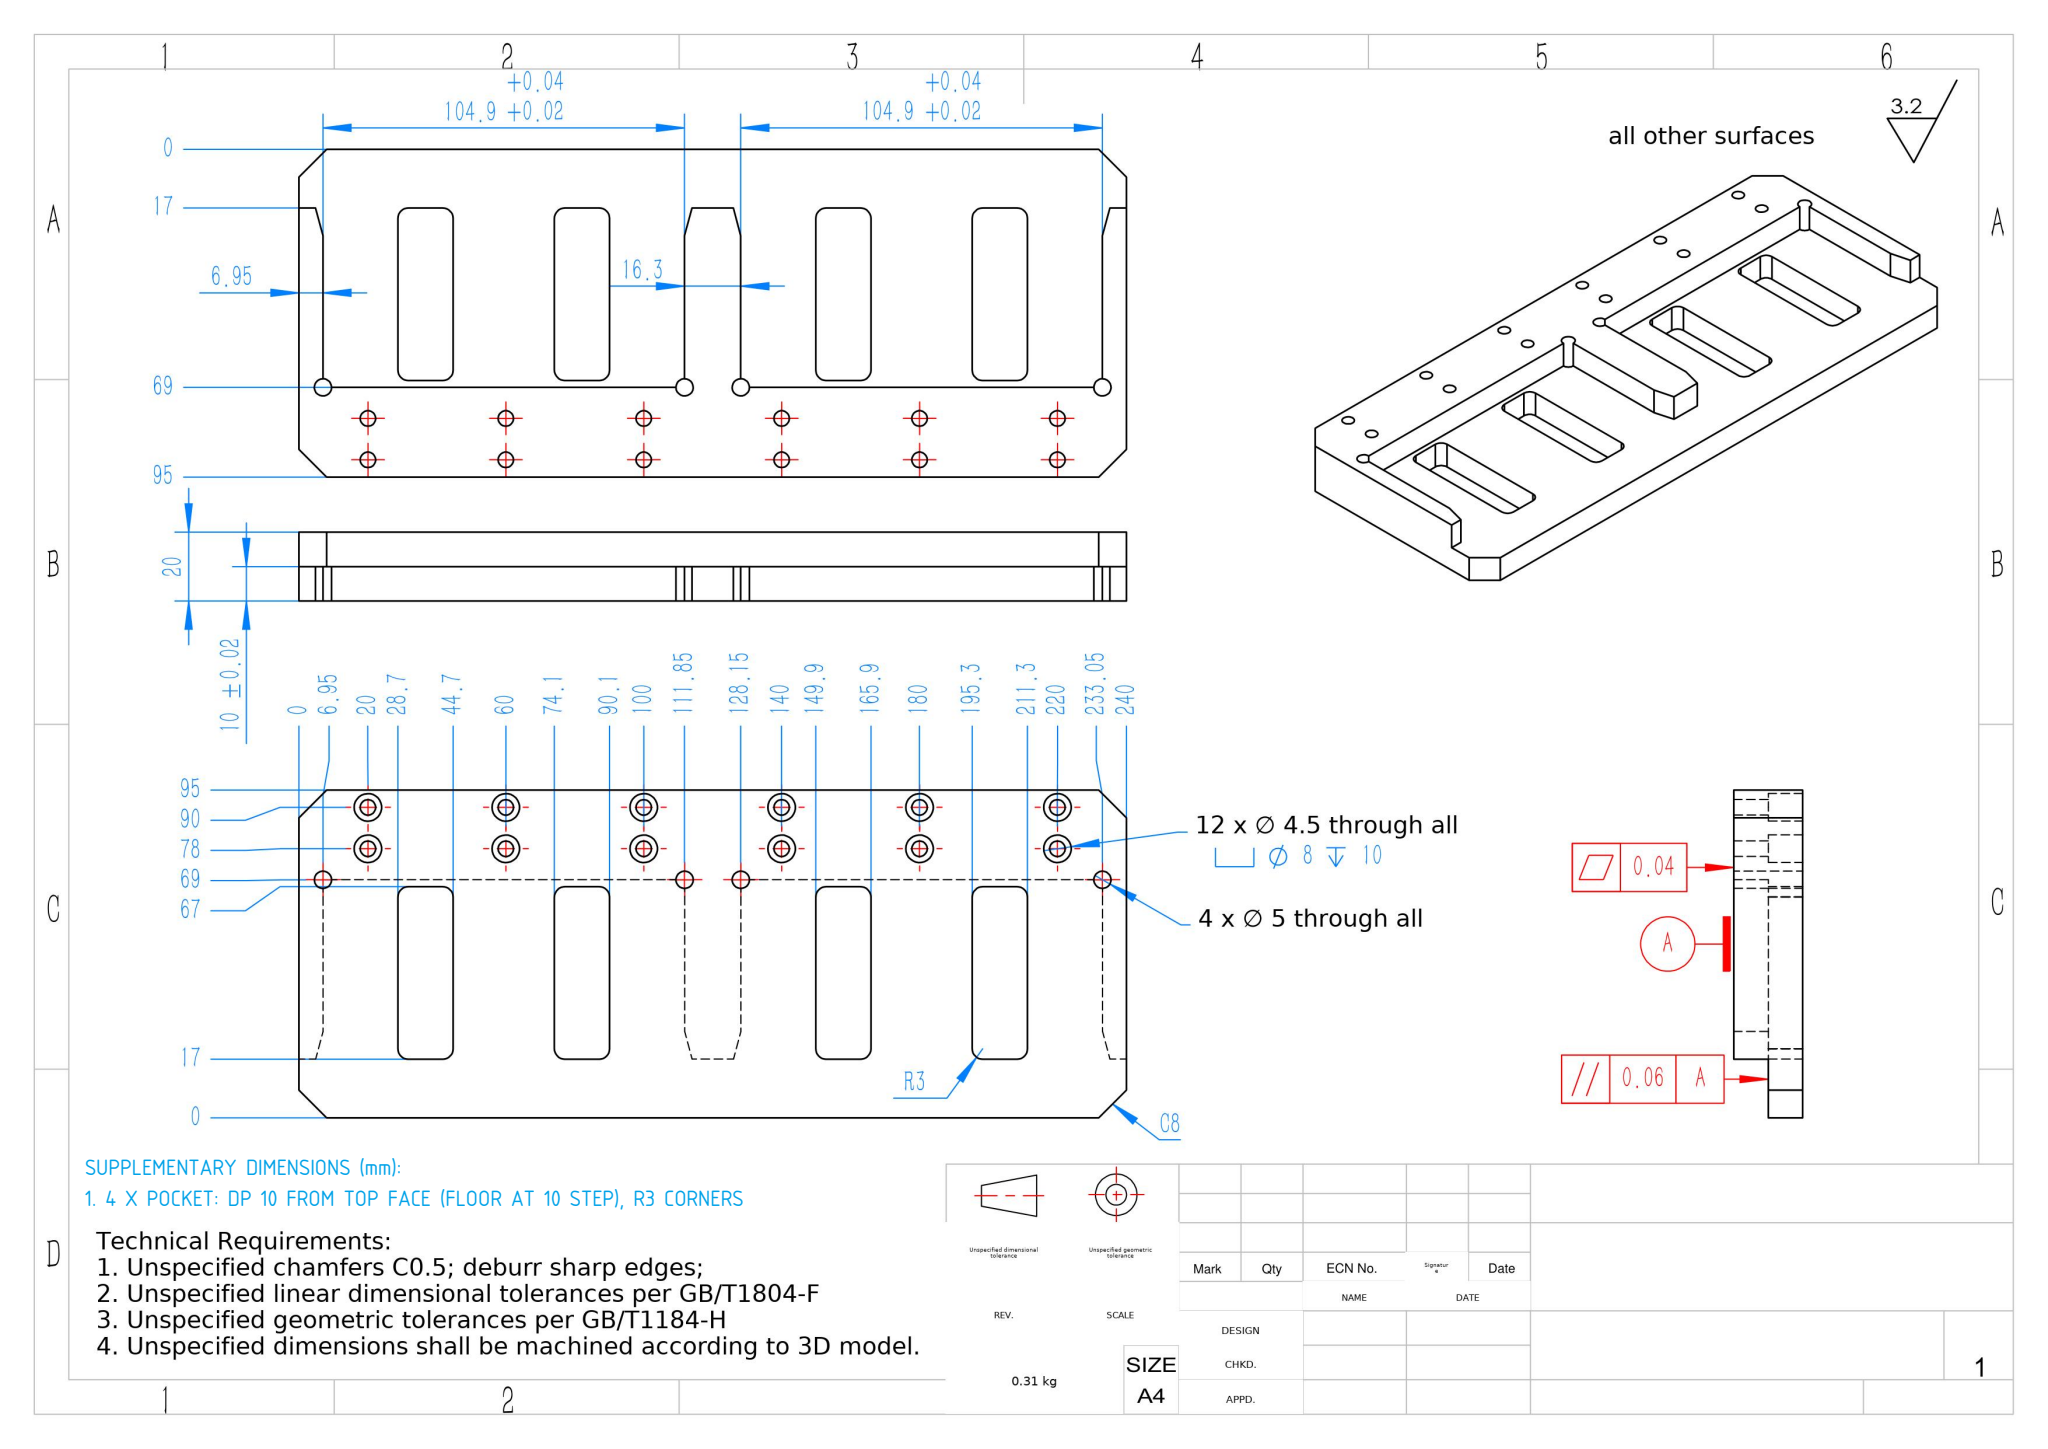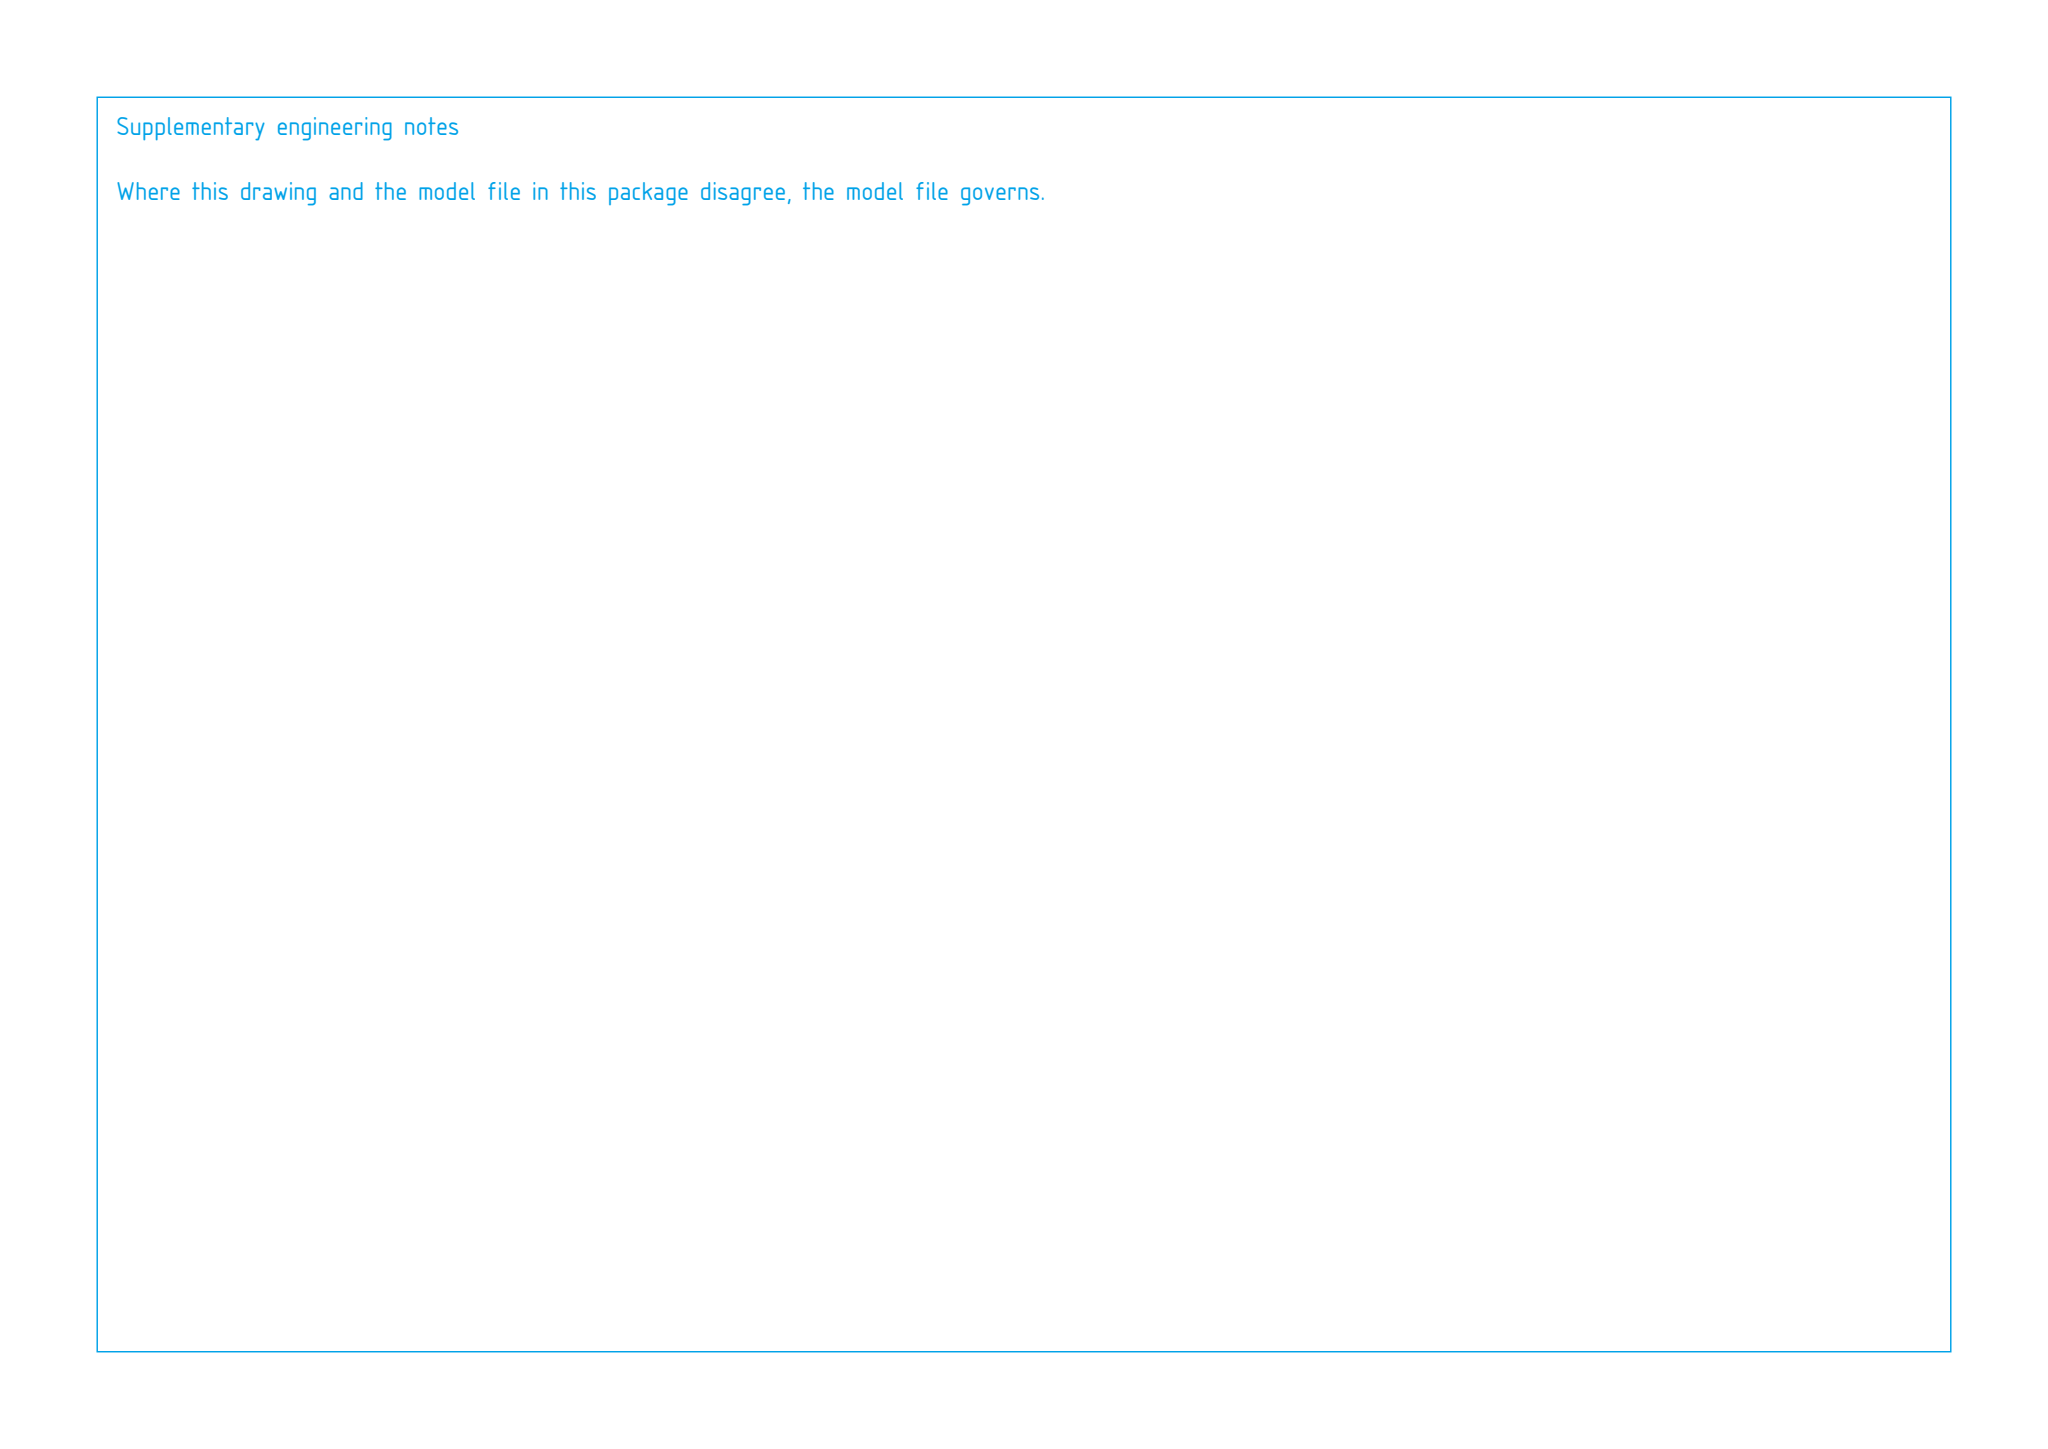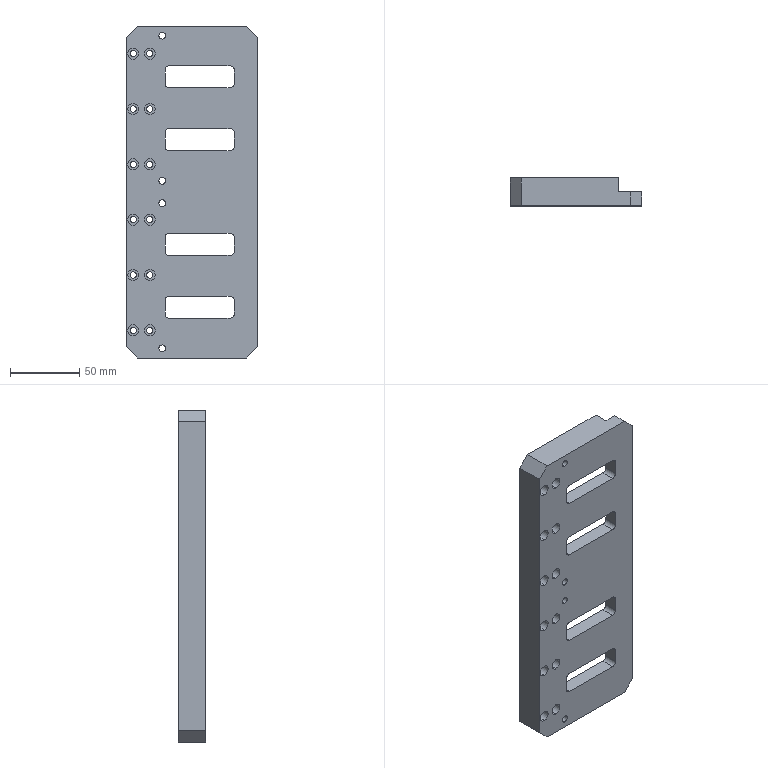Part | SolidWorks | mm | 1 solid | 124 faces | box 95 x 20 x 240 mm | volume 262835 mm3 | cylinder 72 | plane 52 | commonest cylinder face diameters 8 x24 4.5 x24 6 x16 5 x8
build123d program:
from build123d import *
from OCP.BRepFilletAPI import BRepFilletAPI_MakeChamfer

# Parameters (mm, degrees)
SKETCH2_W                                       = 40
SKETCH2_H                                       = 240
BOSS_EXTRUDE1_DEPTH                             = 5
SKETCH13_W                                      = 26
SKETCH13_H                                      = 240
BOSS_EXTRUDE4_DEPTH                             = 10
SKETCH9_W                                       = 240
SKETCH9_H                                       = 10
BOSS_EXTRUDE3_DEPTH                             = 55
CUT_EXTRUDE3_DEPTH                              = 142.863
CUT_EXTRUDE3_DEPTH_BACK                         = 142.863
SKETCH10_W                                      = 50
SKETCH10_H                                      = 16
SKETCH15_W                                      = 52
SKETCH15_H                                      = 16.3
SKETCH15_H_2                                    = 6.95
BOSS_EXTRUDE5_DEPTH                             = 10
CHAMFER1_SIZE                                   = 8
CHAMFER1_SIZE2                                  = 2.144
CHAMFER2_SIZE                                   = 8
CHAMFER2_SIZE2                                  = 2.144
F_5_0_5_DIAMETER_HOLE1_D                        = 5
M4_HEX_SOCKET_HEAD_CAP_SCREW_CBORE1_D           = 4.5
M4_HEX_SOCKET_HEAD_CAP_SCREW_CBORE1_CBORE_D     = 8
M4_HEX_SOCKET_HEAD_CAP_SCREW_CBORE1_CBORE_DEPTH = 10
CHAMFER3_SIZE                                   = 8
FILLET1_R                                       = 3


with BuildPart() as part:
    # Sketch2 → Boss-Extrude1 (new, symmetric)
    with BuildSketch(Plane(origin=(0, 0, 0), x_dir=(1, 0, 0), z_dir=(0, 1, 0))):
        Rectangle(SKETCH2_W, SKETCH2_H)
    extrude(amount=BOSS_EXTRUDE1_DEPTH, both=True)

    # Sketch13 → Boss-Extrude4 (add)
    with BuildSketch(Plane(origin=(0, 5, 0), x_dir=(1, 0, 0), z_dir=(0, 1, 0))):
        with Locations((-7, 0)):
            Rectangle(SKETCH13_W, SKETCH13_H)
    extrude(amount=BOSS_EXTRUDE4_DEPTH)

    # Sketch9 → Boss-Extrude3 (add)
    with BuildSketch(Plane(origin=(20, 0, 0), x_dir=(0, 0, -1), z_dir=(1, 0, 0))):
        Rectangle(SKETCH9_W, SKETCH9_H)
    extrude(amount=BOSS_EXTRUDE3_DEPTH)

    # Sketch10 → Cut-Extrude3 (cut, two sides: drawn at the far end of the back side and taken through both)
    with BuildSketch(Plane(origin=(0, 5, 0), x_dir=(1, 0, 0), z_dir=(0, 1, 0)).offset(-CUT_EXTRUDE3_DEPTH_BACK)):
        with Locations((33, 83.3)):
            Rectangle(SKETCH10_W, SKETCH10_H)
        with Locations((33, 37.9)):
            Rectangle(SKETCH10_W, SKETCH10_H)
        with Locations((33, -37.9)):
            Rectangle(SKETCH10_W, SKETCH10_H)
        with Locations((33, -83.3)):
            Rectangle(SKETCH10_W, SKETCH10_H)
    extrude(amount=CUT_EXTRUDE3_DEPTH + CUT_EXTRUDE3_DEPTH_BACK, mode=Mode.SUBTRACT)

    # Sketch15 → Boss-Extrude5 (add)
    with BuildSketch(Plane(origin=(0, 5, 0), x_dir=(1, 0, 0), z_dir=(0, 1, 0))):
        with Locations((32, 0)):
            Rectangle(SKETCH15_W, SKETCH15_H)
        with Locations((32, 116.525)):
            Rectangle(SKETCH15_W, SKETCH15_H_2)
        with Locations((32, -116.525)):
            Rectangle(SKETCH15_W, SKETCH15_H_2)
    extrude(amount=BOSS_EXTRUDE5_DEPTH)

    # Chamfer1: one chamfer whose edges measure the first distance from different faces: ONE call of the kernel's chamfer builder (chamfer() names one face for all edges)
    chamfer1_edges_1 = [part.edges().sort_by_distance(p)[0] for p in [
        (58, 10, 8.15),
    ]]
    chamfer1_side_1 = [part.faces().sort_by_distance(p)[0] for p in [
        (32, 10, 8.15),
    ]]
    chamfer1_edges_2 = [part.edges().sort_by_distance(p)[0] for p in [
        (58, 10, -113.05),
    ]]
    chamfer1_side_2 = [part.faces().sort_by_distance(p)[0] for p in [
        (32, 10, -113.05),
    ]]
    chamfer1 = BRepFilletAPI_MakeChamfer(part.part.solid().wrapped)
    for e in chamfer1_edges_1:
        chamfer1.Add(CHAMFER1_SIZE, CHAMFER1_SIZE2, e.wrapped, chamfer1_side_1[0].wrapped)  # the first distance lies on this face
    for e in chamfer1_edges_2:
        chamfer1.Add(CHAMFER1_SIZE, CHAMFER1_SIZE2, e.wrapped, chamfer1_side_2[0].wrapped)  # the first distance lies on this face
    add(Compound.cast(chamfer1.Shape()), mode=Mode.REPLACE)

    # Chamfer2: one chamfer whose edges measure the first distance from different faces: ONE call of the kernel's chamfer builder (chamfer() names one face for all edges)
    chamfer2_edges_1 = [part.edges().sort_by_distance(p)[0] for p in [
        (58, 10, -8.15),
    ]]
    chamfer2_side_1 = [part.faces().sort_by_distance(p)[0] for p in [
        (32, 10, -8.15),
    ]]
    chamfer2_edges_2 = [part.edges().sort_by_distance(p)[0] for p in [
        (58, 10, 113.05),
    ]]
    chamfer2_side_2 = [part.faces().sort_by_distance(p)[0] for p in [
        (32, 10, 113.05),
    ]]
    chamfer2 = BRepFilletAPI_MakeChamfer(part.part.solid().wrapped)
    for e in chamfer2_edges_1:
        chamfer2.Add(CHAMFER2_SIZE, CHAMFER2_SIZE2, e.wrapped, chamfer2_side_1[0].wrapped)  # the first distance lies on this face
    for e in chamfer2_edges_2:
        chamfer2.Add(CHAMFER2_SIZE, CHAMFER2_SIZE2, e.wrapped, chamfer2_side_2[0].wrapped)  # the first distance lies on this face
    add(Compound.cast(chamfer2.Shape()), mode=Mode.REPLACE)

    # 5.0 _5_ Diameter Hole1 (through all)
    with Locations(Plane(origin=(0, 15, 0), x_dir=(1, 0, 0), z_dir=(0, 1, 0))):
        with Locations((6, -113.05), (6, -8.15), (6, 8.15), (6, 113.05)):
            Hole(F_5_0_5_DIAMETER_HOLE1_D / 2)

    # M4 Hex Socket Head Cap Screw CBORE1 (through all)
    with Locations(Plane(origin=(0, -5, 0), x_dir=(-1, 0, 0), z_dir=(0, -1, 0))):
        with Locations((15, -100), (3, -100), (3, -60), (15, -60), (15, -20), (3, -20), (3, 20), (15, 20), (15, 60), (3, 60), (3, 100), (15, 100)):
            CounterBoreHole(M4_HEX_SOCKET_HEAD_CAP_SCREW_CBORE1_D / 2, M4_HEX_SOCKET_HEAD_CAP_SCREW_CBORE1_CBORE_D / 2, M4_HEX_SOCKET_HEAD_CAP_SCREW_CBORE1_CBORE_DEPTH)

    # Chamfer3
    chamfer3_edges = [part.edges().sort_by_distance(p)[0] for p in [
        (75, 0, 120),
        (75, 0, -120),
        (-20, 5, 120),
        (-20, 5, -120),
    ]]
    chamfer(chamfer3_edges, length=CHAMFER3_SIZE)

    # Fillet1
    fillet1_edges = [part.edges().sort_by_distance(p)[0] for p in [
        (58, 0, -91.3),
        (58, 0, -75.3),
        (8, 0, -75.3),
        (8, 0, -91.3),
        (8, 0, -29.9),
        (8, 0, -45.9),
        (58, 0, -45.9),
        (58, 0, -29.9),
        (8, 0, 45.9),
        (8, 0, 29.9),
        (58, 0, 29.9),
        (58, 0, 45.9),
        (8, 0, 91.3),
        (8, 0, 75.3),
        (58, 0, 75.3),
        (58, 0, 91.3),
    ]]
    fillet(fillet1_edges, radius=FILLET1_R)


solid = part.part